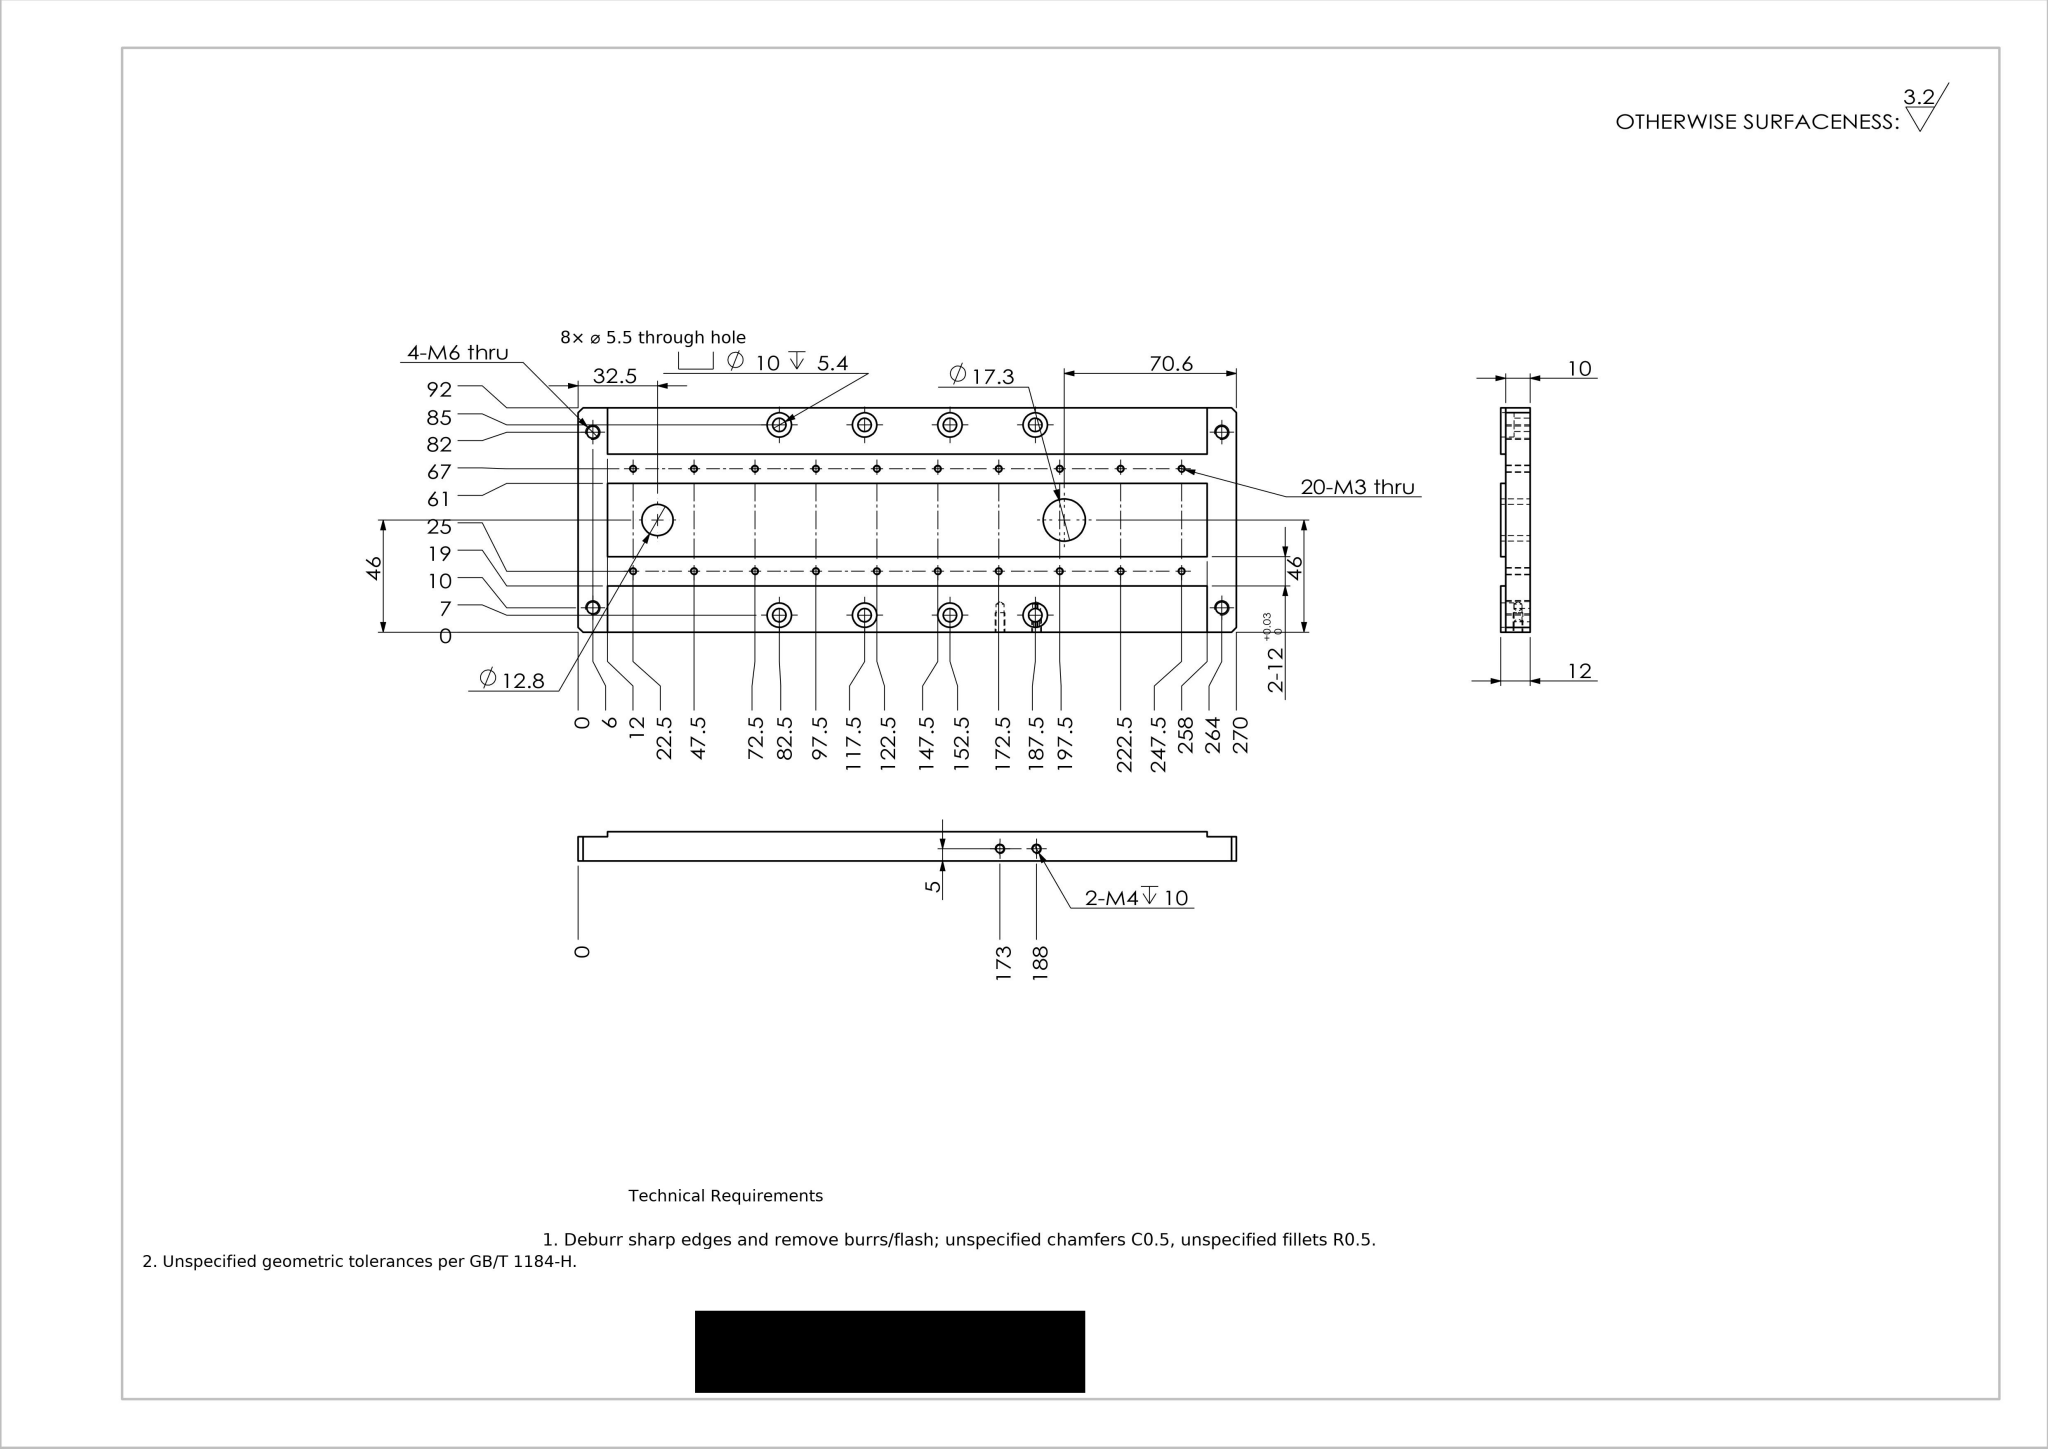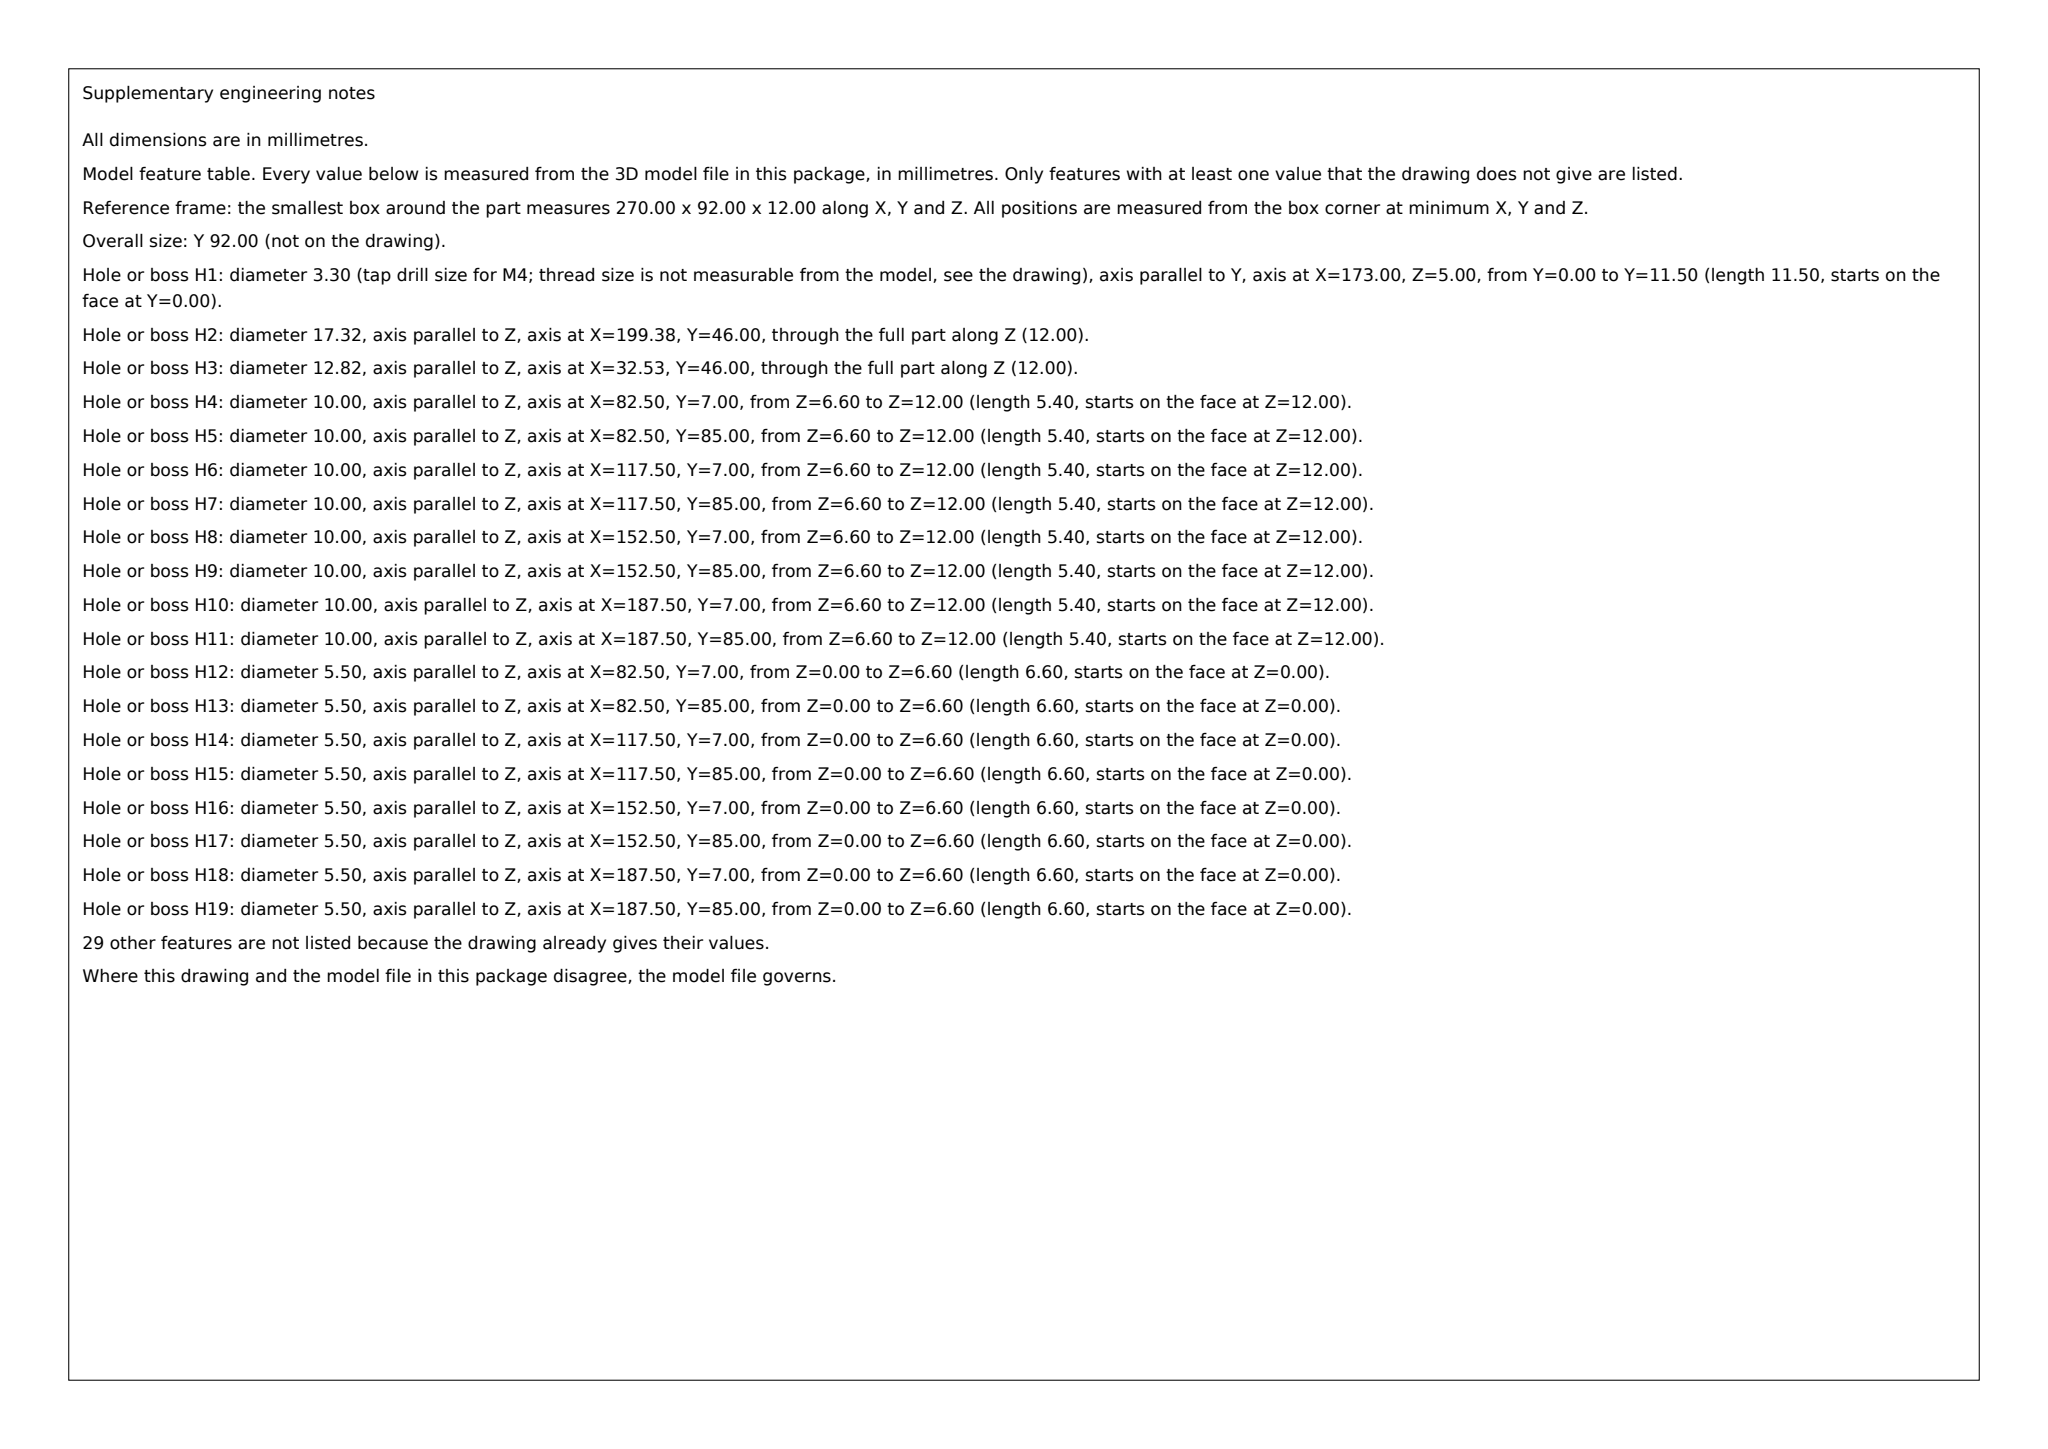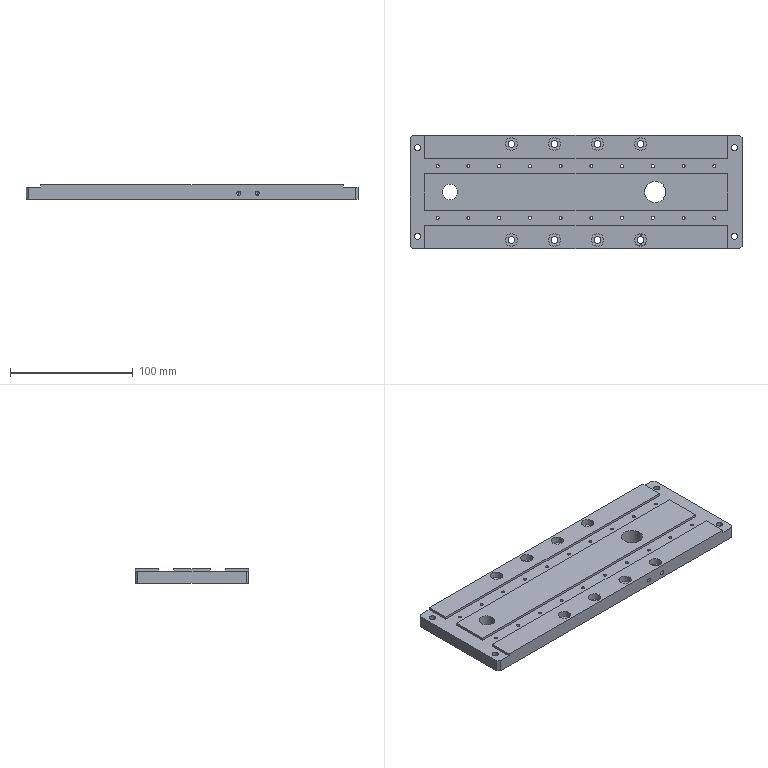Part | SolidWorks | mm | 1 solid | 125 faces | box 270 x 92 x 12 mm | volume 270827 mm3 | cylinder 90 | plane 31 | cone 4 | commonest cylinder face diameters 2.5 x40 10 x16 5.5 x16 5 x8 3.3 x6 12.828 x2 17.314 x2
build123d program:
from build123d import *

# Parameters (mm, degrees)
SKETCH1_W                                       = 270
SKETCH1_H                                       = 92
BOSS_EXTRUDE1_DEPTH                             = 12
SKETCH2_W                                       = 270
SKETCH2_H                                       = 12
CUT_EXTRUDE1_DEPTH                              = 2
SKETCH3_W                                       = 12
SKETCH3_H                                       = 92
CUT_EXTRUDE2_DEPTH                              = 2
CHAMFER1_SIZE                                   = 2
M6_TAPPED_HOLE1_D                               = 5
M5_HEX_SOCKET_HEAD_CAP_SCREW_CBORE1_D           = 5.5
M5_HEX_SOCKET_HEAD_CAP_SCREW_CBORE1_CBORE_D     = 10
M5_HEX_SOCKET_HEAD_CAP_SCREW_CBORE1_CBORE_DEPTH = 5.4
M3_TAPPED_HOLE2_D                               = 2.5
LPATTERN1_COUNT                                 = 10
LPATTERN1_PITCH                                 = 25
LPATTERN1_COUNT_DIR2                            = 2
LPATTERN1_PITCH_DIR2                            = 42
M4_TAPPED_HOLE1_D                               = 3.3
M4_TAPPED_HOLE1_DEPTH                           = 11.5
M4_TAPPED_HOLE1_TIP                             = 0.9914
SKETCH18_R                                      = 6.414
SKETCH18_R_2                                    = 8.657
CUT_EXTRUDE3_DEPTH                              = 80


with BuildPart() as part:
    # Sketch1 → Boss-Extrude1 (new body)
    with BuildSketch(Plane.XY):
        Rectangle(SKETCH1_W, SKETCH1_H)
    extrude(amount=BOSS_EXTRUDE1_DEPTH)

    # Sketch2 → Cut-Extrude1 (cut)
    with BuildSketch(Plane.XY.offset(12)):
        with Locations((0, -21)):
            Rectangle(SKETCH2_W, SKETCH2_H)
        with Locations((0, 21)):
            Rectangle(SKETCH2_W, SKETCH2_H)
    extrude(amount=-CUT_EXTRUDE1_DEPTH, mode=Mode.SUBTRACT)

    # Sketch3 → Cut-Extrude2 (cut)
    with BuildSketch(Plane.XY.offset(12)):
        with Locations((-129, 0)):
            Rectangle(SKETCH3_W, SKETCH3_H)
        with Locations((129, 0)):
            Rectangle(SKETCH3_W, SKETCH3_H)
    extrude(amount=-CUT_EXTRUDE2_DEPTH, mode=Mode.SUBTRACT)

    # Chamfer1
    chamfer1_edges = [part.edges().sort_by_distance(p)[0] for p in [
        (-135, -46, 5),
        (-135, 46, 5),
        (135, -46, 5),
        (135, 46, 5),
    ]]
    chamfer(chamfer1_edges, length=CHAMFER1_SIZE)

    # M6 Tapped Hole1 (through all)
    with Locations(Plane.XY.offset(10)):
        with Locations((-129, 36), (-129, -36), (129, 36), (129, -36)):
            Hole(M6_TAPPED_HOLE1_D / 2)

    # M5 Hex Socket Head Cap Screw CBORE1 (through all)
    with Locations(Plane.XY.offset(12)):
        with Locations((-52.5, 39), (-17.5, 39), (52.5, 39), (52.5, -39), (-17.5, -39), (-52.5, -39), (17.5, 39), (17.5, -39)):
            CounterBoreHole(M5_HEX_SOCKET_HEAD_CAP_SCREW_CBORE1_D / 2, M5_HEX_SOCKET_HEAD_CAP_SCREW_CBORE1_CBORE_D / 2, M5_HEX_SOCKET_HEAD_CAP_SCREW_CBORE1_CBORE_DEPTH)

    # M3 Tapped Hole2 (through all)
    with Locations(Plane.XY.offset(10)):
        with Locations((112.5, -21)):
            m3_tapped_hole2 = Hole(M3_TAPPED_HOLE2_D / 2)

    # LPattern1: M3 Tapped Hole2 10 × 2
    with Locations(*[(-i * LPATTERN1_PITCH, j * LPATTERN1_PITCH_DIR2, 0) for i in range(LPATTERN1_COUNT) for j in range(LPATTERN1_COUNT_DIR2) if (i, j) != (0, 0)]):
        add(m3_tapped_hole2, mode=Mode.SUBTRACT)

    # M4 Tapped Hole1
    with Locations(Plane(origin=(6.717, -46, -0.5978), x_dir=(1, 0, 0), z_dir=(0, -1, 0))):
        with Locations((46.283, 5.598), (31.283, 5.598)):
            Hole(M4_TAPPED_HOLE1_D / 2, depth=M4_TAPPED_HOLE1_DEPTH)
            with Locations((0, 0, -(M4_TAPPED_HOLE1_DEPTH + M4_TAPPED_HOLE1_TIP / 2))):  # 118° drill point
                Cone(0, M4_TAPPED_HOLE1_D / 2, M4_TAPPED_HOLE1_TIP, mode=Mode.SUBTRACT)

    # Sketch18 → Cut-Extrude3 (cut)
    with BuildSketch(Plane.XY.offset(12)):
        with Locations((-102.468, 0)):
            Circle(SKETCH18_R)
        with Locations((64.382, 0)):
            Circle(SKETCH18_R_2)
    extrude(amount=-CUT_EXTRUDE3_DEPTH, mode=Mode.SUBTRACT)


solid = part.part